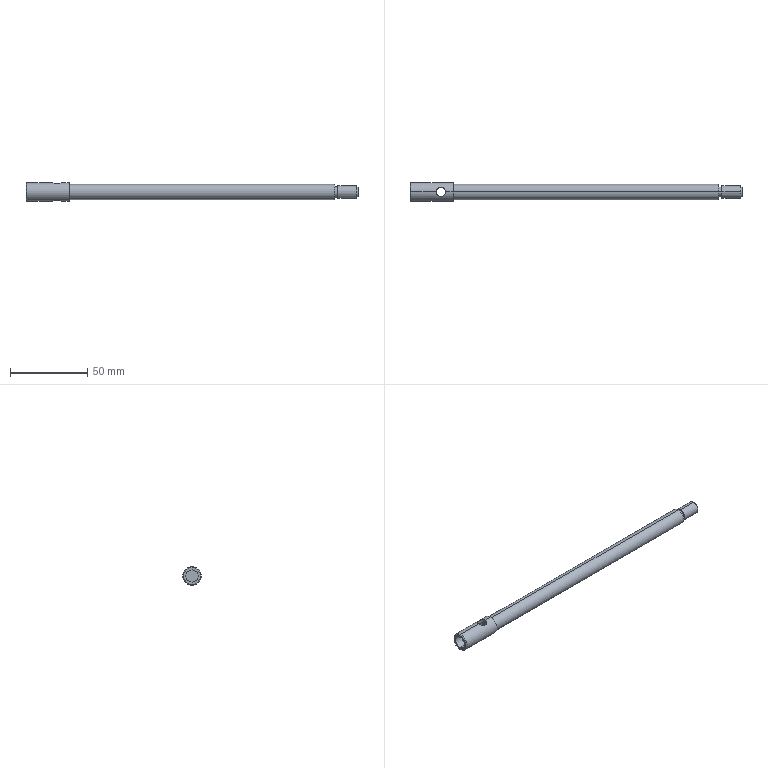Component | SolidWorks | Barrel-1 | 1 solid | 27 faces | box 215 x 12 x 12 mm | volume 14334 mm3 | cylinder 16 | plane 7 | cone 4 | commonest cylinder face diameters 6 x4 8 x4 5 x2 6.5 x2 10 x2 12 x2
STEP:
#1=CARTESIAN_POINT('',(-16.568,1.358,39.941));
#2=VERTEX_POINT('',#1);
#3=CARTESIAN_POINT('',(-16.568,1.358,39.508));
#4=VERTEX_POINT('',#3);
#5=CARTESIAN_POINT('',(-16.568,1.358,39.724));
#6=DIRECTION('',(-1.,0.,0.));
#7=DIRECTION('',(0.,0.,-1.));
#8=AXIS2_PLACEMENT_3D('',#5,#6,#7);
#9=CIRCLE('',#8,0.2165);
#10=EDGE_CURVE('',#2,#4,#9,.T.);
#11=ORIENTED_EDGE('',*,*,#10,.F.);
#12=CARTESIAN_POINT('',(-16.548,1.358,39.961));
#13=VERTEX_POINT('',#12);
#14=CARTESIAN_POINT('',(-16.568,1.358,39.941));
#15=DIRECTION('',(0.7071,0.,0.7071));
#16=VECTOR('',#15,39.37);
#17=LINE('',#14,#16);
#18=EDGE_CURVE('',#2,#13,#17,.T.);
#19=ORIENTED_EDGE('',*,*,#18,.T.);
#20=CARTESIAN_POINT('',(-16.548,1.358,39.488));
#21=VERTEX_POINT('',#20);
#22=CARTESIAN_POINT('',(-16.548,1.358,39.724));
#23=DIRECTION('',(1.,0.,0.));
#24=DIRECTION('',(0.,0.,-1.));
#25=AXIS2_PLACEMENT_3D('',#22,#23,#24);
#26=CIRCLE('',#25,0.2362);
#27=EDGE_CURVE('',#21,#13,#26,.T.);
#28=ORIENTED_EDGE('',*,*,#27,.F.);
#29=CARTESIAN_POINT('',(-16.568,1.358,39.508));
#30=DIRECTION('',(0.7071,0.,-0.7071));
#31=VECTOR('',#30,39.37);
#32=LINE('',#29,#31);
#33=EDGE_CURVE('',#4,#21,#32,.T.);
#34=ORIENTED_EDGE('',*,*,#33,.F.);
#35=EDGE_LOOP('',(#11,#19,#28,#34));
#36=FACE_OUTER_BOUND('',#35,.T.);
#37=CARTESIAN_POINT('',(-16.568,1.358,39.724));
#38=DIRECTION('',(1.,0.,0.));
#39=DIRECTION('',(0.,0.,-1.));
#40=AXIS2_PLACEMENT_3D('',#37,#38,#39);
#41=CONICAL_SURFACE('',#40,0.2165,0.7854);
#42=ADVANCED_FACE('',(#36),#41,.T.);
#43=CARTESIAN_POINT('',(-15.898,1.358,39.961));
#44=VERTEX_POINT('',#43);
#45=CARTESIAN_POINT('',(-15.662,1.358,39.961));
#46=VERTEX_POINT('',#45);
#47=CARTESIAN_POINT('',(-15.898,1.358,39.961));
#48=CARTESIAN_POINT('',(-15.898,1.35,39.961));
#49=CARTESIAN_POINT('',(-15.898,1.342,39.96));
#50=CARTESIAN_POINT('',(-15.894,1.326,39.959));
#51=CARTESIAN_POINT('',(-15.892,1.319,39.958));
#52=CARTESIAN_POINT('',(-15.886,1.305,39.955));
#53=CARTESIAN_POINT('',(-15.882,1.298,39.953));
#54=CARTESIAN_POINT('',(-15.874,1.285,39.949));
#55=CARTESIAN_POINT('',(-15.869,1.279,39.947));
#56=CARTESIAN_POINT('',(-15.858,1.269,39.943));
#57=CARTESIAN_POINT('',(-15.852,1.264,39.941));
#58=CARTESIAN_POINT('',(-15.84,1.255,39.937));
#59=CARTESIAN_POINT('',(-15.833,1.252,39.936));
#60=CARTESIAN_POINT('',(-15.819,1.246,39.932));
#61=CARTESIAN_POINT('',(-15.811,1.243,39.931));
#62=CARTESIAN_POINT('',(-15.796,1.24,39.929));
#63=CARTESIAN_POINT('',(-15.788,1.239,39.929));
#64=CARTESIAN_POINT('',(-15.773,1.239,39.929));
#65=CARTESIAN_POINT('',(-15.765,1.24,39.929));
#66=CARTESIAN_POINT('',(-15.749,1.243,39.931));
#67=CARTESIAN_POINT('',(-15.742,1.246,39.932));
#68=CARTESIAN_POINT('',(-15.72,1.255,39.937));
#69=CARTESIAN_POINT('',(-15.708,1.263,39.941));
#70=CARTESIAN_POINT('',(-15.691,1.279,39.947));
#71=CARTESIAN_POINT('',(-15.687,1.285,39.949));
#72=CARTESIAN_POINT('',(-15.678,1.298,39.953));
#73=CARTESIAN_POINT('',(-15.674,1.305,39.955));
#74=CARTESIAN_POINT('',(-15.668,1.319,39.958));
#75=CARTESIAN_POINT('',(-15.666,1.326,39.959));
#76=CARTESIAN_POINT('',(-15.663,1.342,39.96));
#77=CARTESIAN_POINT('',(-15.662,1.35,39.961));
#78=CARTESIAN_POINT('',(-15.662,1.358,39.961));
#79=B_SPLINE_CURVE_WITH_KNOTS('',3,(#47,#48,#49,#50,#51,#52,#53,#54,#55,#56,#57,#58,#59,#60,#61,#62,#63,#64,#65,#66,#67,#68,#69,#70,#71,#72,#73,#74,#75,#76,#77,#78),.UNSPECIFIED.,.F.,.F.,(4,2,2,2,2,2,2,2,2,2,2,2,2,2,2,4),(0.009543,0.01014,0.01073,0.01133,0.01192,0.01252,0.01312,0.01371,0.01431,0.0149,0.0155,0.01669,0.01728,0.01788,0.01847,0.01907),.UNSPECIFIED.);
#80=EDGE_CURVE('',#44,#46,#79,.T.);
#81=ORIENTED_EDGE('',*,*,#80,.T.);
#82=CARTESIAN_POINT('',(-15.662,1.358,39.882));
#83=VERTEX_POINT('',#82);
#84=CARTESIAN_POINT('',(-15.662,1.358,40.472));
#85=DIRECTION('',(0.,0.,-1.));
#86=VECTOR('',#85,39.37);
#87=LINE('',#84,#86);
#88=EDGE_CURVE('',#46,#83,#87,.T.);
#89=ORIENTED_EDGE('',*,*,#88,.T.);
#90=CARTESIAN_POINT('',(-15.898,1.358,39.882));
#91=VERTEX_POINT('',#90);
#92=CARTESIAN_POINT('',(-15.662,1.358,39.882));
#93=CARTESIAN_POINT('',(-15.662,1.349,39.882));
#94=CARTESIAN_POINT('',(-15.663,1.341,39.881));
#95=CARTESIAN_POINT('',(-15.666,1.326,39.879));
#96=CARTESIAN_POINT('',(-15.669,1.318,39.877));
#97=CARTESIAN_POINT('',(-15.675,1.304,39.873));
#98=CARTESIAN_POINT('',(-15.679,1.297,39.87));
#99=CARTESIAN_POINT('',(-15.687,1.285,39.864));
#100=CARTESIAN_POINT('',(-15.692,1.279,39.861));
#101=CARTESIAN_POINT('',(-15.702,1.268,39.854));
#102=CARTESIAN_POINT('',(-15.708,1.264,39.851));
#103=CARTESIAN_POINT('',(-15.72,1.255,39.844));
#104=CARTESIAN_POINT('',(-15.727,1.252,39.841));
#105=CARTESIAN_POINT('',(-15.741,1.246,39.836));
#106=CARTESIAN_POINT('',(-15.748,1.244,39.833));
#107=CARTESIAN_POINT('',(-15.764,1.24,39.83));
#108=CARTESIAN_POINT('',(-15.772,1.239,39.829));
#109=CARTESIAN_POINT('',(-15.788,1.239,39.829));
#110=CARTESIAN_POINT('',(-15.796,1.24,39.83));
#111=CARTESIAN_POINT('',(-15.812,1.244,39.833));
#112=CARTESIAN_POINT('',(-15.819,1.246,39.836));
#113=CARTESIAN_POINT('',(-15.833,1.252,39.841));
#114=CARTESIAN_POINT('',(-15.84,1.255,39.844));
#115=CARTESIAN_POINT('',(-15.852,1.264,39.851));
#116=CARTESIAN_POINT('',(-15.858,1.268,39.854));
#117=CARTESIAN_POINT('',(-15.869,1.279,39.861));
#118=CARTESIAN_POINT('',(-15.873,1.285,39.864));
#119=CARTESIAN_POINT('',(-15.882,1.297,39.87));
#120=CARTESIAN_POINT('',(-15.886,1.304,39.873));
#121=CARTESIAN_POINT('',(-15.892,1.318,39.877));
#122=CARTESIAN_POINT('',(-15.894,1.326,39.879));
#123=CARTESIAN_POINT('',(-15.898,1.342,39.881));
#124=CARTESIAN_POINT('',(-15.898,1.35,39.882));
#125=CARTESIAN_POINT('',(-15.898,1.358,39.882));
#126=B_SPLINE_CURVE_WITH_KNOTS('',3,(#92,#93,#94,#95,#96,#97,#98,#99,#100,#101,#102,#103,#104,#105,#106,#107,#108,#109,#110,#111,#112,#113,#114,#115,#116,#117,#118,#119,#120,#121,#122,#123,#124,#125),.UNSPECIFIED.,.F.,.F.,(4,2,2,2,2,2,2,2,2,2,2,2,2,2,2,2,4),(0.,0.0006141,0.001228,0.001842,0.002456,0.003071,0.003685,0.004299,0.004913,0.005527,0.006141,0.006755,0.007369,0.007983,0.008598,0.009212,0.009826),.UNSPECIFIED.);
#127=EDGE_CURVE('',#83,#91,#126,.T.);
#128=ORIENTED_EDGE('',*,*,#127,.T.);
#129=CARTESIAN_POINT('',(-15.898,1.358,40.472));
#130=DIRECTION('',(0.,0.,-1.));
#131=VECTOR('',#130,39.37);
#132=LINE('',#129,#131);
#133=EDGE_CURVE('',#44,#91,#132,.T.);
#134=ORIENTED_EDGE('',*,*,#133,.F.);
#135=EDGE_LOOP('',(#81,#89,#128,#134));
#136=FACE_OUTER_BOUND('',#135,.T.);
#137=CARTESIAN_POINT('',(-15.78,1.358,40.472));
#138=DIRECTION('',(0.,0.,-1.));
#139=DIRECTION('',(-1.,0.,0.));
#140=AXIS2_PLACEMENT_3D('',#137,#138,#139);
#141=CYLINDRICAL_SURFACE('',#140,0.1181);
#142=ADVANCED_FACE('',(#136),#141,.F.);
#143=CARTESIAN_POINT('',(-15.898,1.358,39.567));
#144=VERTEX_POINT('',#143);
#145=CARTESIAN_POINT('',(-15.662,1.358,39.567));
#146=VERTEX_POINT('',#145);
#147=CARTESIAN_POINT('',(-15.898,1.358,39.567));
#148=CARTESIAN_POINT('',(-15.898,1.349,39.567));
#149=CARTESIAN_POINT('',(-15.897,1.341,39.568));
#150=CARTESIAN_POINT('',(-15.894,1.326,39.57));
#151=CARTESIAN_POINT('',(-15.892,1.318,39.572));
#152=CARTESIAN_POINT('',(-15.886,1.304,39.576));
#153=CARTESIAN_POINT('',(-15.882,1.297,39.579));
#154=CARTESIAN_POINT('',(-15.873,1.285,39.585));
#155=CARTESIAN_POINT('',(-15.869,1.279,39.588));
#156=CARTESIAN_POINT('',(-15.858,1.268,39.594));
#157=CARTESIAN_POINT('',(-15.852,1.264,39.598));
#158=CARTESIAN_POINT('',(-15.84,1.255,39.604));
#159=CARTESIAN_POINT('',(-15.833,1.252,39.608));
#160=CARTESIAN_POINT('',(-15.819,1.246,39.613));
#161=CARTESIAN_POINT('',(-15.812,1.244,39.616));
#162=CARTESIAN_POINT('',(-15.796,1.24,39.619));
#163=CARTESIAN_POINT('',(-15.788,1.239,39.62));
#164=CARTESIAN_POINT('',(-15.772,1.239,39.62));
#165=CARTESIAN_POINT('',(-15.764,1.24,39.619));
#166=CARTESIAN_POINT('',(-15.748,1.244,39.616));
#167=CARTESIAN_POINT('',(-15.741,1.246,39.613));
#168=CARTESIAN_POINT('',(-15.727,1.252,39.608));
#169=CARTESIAN_POINT('',(-15.72,1.255,39.604));
#170=CARTESIAN_POINT('',(-15.708,1.264,39.598));
#171=CARTESIAN_POINT('',(-15.702,1.268,39.594));
#172=CARTESIAN_POINT('',(-15.692,1.279,39.588));
#173=CARTESIAN_POINT('',(-15.687,1.285,39.585));
#174=CARTESIAN_POINT('',(-15.679,1.297,39.579));
#175=CARTESIAN_POINT('',(-15.675,1.304,39.576));
#176=CARTESIAN_POINT('',(-15.669,1.318,39.572));
#177=CARTESIAN_POINT('',(-15.666,1.326,39.57));
#178=CARTESIAN_POINT('',(-15.663,1.342,39.568));
#179=CARTESIAN_POINT('',(-15.662,1.35,39.567));
#180=CARTESIAN_POINT('',(-15.662,1.358,39.567));
#181=B_SPLINE_CURVE_WITH_KNOTS('',3,(#147,#148,#149,#150,#151,#152,#153,#154,#155,#156,#157,#158,#159,#160,#161,#162,#163,#164,#165,#166,#167,#168,#169,#170,#171,#172,#173,#174,#175,#176,#177,#178,#179,#180),.UNSPECIFIED.,.F.,.F.,(4,2,2,2,2,2,2,2,2,2,2,2,2,2,2,2,4),(0.,0.0006141,0.001228,0.001842,0.002456,0.003071,0.003685,0.004299,0.004913,0.005527,0.006141,0.006755,0.007369,0.007983,0.008598,0.009212,0.009826),.UNSPECIFIED.);
#182=EDGE_CURVE('',#144,#146,#181,.T.);
#183=ORIENTED_EDGE('',*,*,#182,.T.);
#184=CARTESIAN_POINT('',(-15.662,1.358,39.488));
#185=VERTEX_POINT('',#184);
#186=CARTESIAN_POINT('',(-15.662,1.358,40.472));
#187=DIRECTION('',(0.,0.,-1.));
#188=VECTOR('',#187,39.37);
#189=LINE('',#186,#188);
#190=EDGE_CURVE('',#146,#185,#189,.T.);
#191=ORIENTED_EDGE('',*,*,#190,.T.);
#192=CARTESIAN_POINT('',(-15.898,1.358,39.488));
#193=VERTEX_POINT('',#192);
#194=CARTESIAN_POINT('',(-15.662,1.358,39.488));
#195=CARTESIAN_POINT('',(-15.662,1.35,39.488));
#196=CARTESIAN_POINT('',(-15.663,1.342,39.489));
#197=CARTESIAN_POINT('',(-15.666,1.326,39.49));
#198=CARTESIAN_POINT('',(-15.668,1.319,39.491));
#199=CARTESIAN_POINT('',(-15.674,1.305,39.494));
#200=CARTESIAN_POINT('',(-15.678,1.298,39.496));
#201=CARTESIAN_POINT('',(-15.687,1.285,39.499));
#202=CARTESIAN_POINT('',(-15.691,1.279,39.501));
#203=CARTESIAN_POINT('',(-15.702,1.269,39.506));
#204=CARTESIAN_POINT('',(-15.708,1.264,39.508));
#205=CARTESIAN_POINT('',(-15.721,1.255,39.511));
#206=CARTESIAN_POINT('',(-15.728,1.252,39.513));
#207=CARTESIAN_POINT('',(-15.742,1.246,39.516));
#208=CARTESIAN_POINT('',(-15.749,1.243,39.518));
#209=CARTESIAN_POINT('',(-15.764,1.24,39.519));
#210=CARTESIAN_POINT('',(-15.772,1.239,39.52));
#211=CARTESIAN_POINT('',(-15.788,1.239,39.52));
#212=CARTESIAN_POINT('',(-15.796,1.24,39.519));
#213=CARTESIAN_POINT('',(-15.811,1.243,39.518));
#214=CARTESIAN_POINT('',(-15.819,1.246,39.516));
#215=CARTESIAN_POINT('',(-15.84,1.255,39.512));
#216=CARTESIAN_POINT('',(-15.853,1.263,39.508));
#217=CARTESIAN_POINT('',(-15.869,1.279,39.501));
#218=CARTESIAN_POINT('',(-15.874,1.285,39.499));
#219=CARTESIAN_POINT('',(-15.882,1.298,39.496));
#220=CARTESIAN_POINT('',(-15.886,1.305,39.494));
#221=CARTESIAN_POINT('',(-15.892,1.319,39.491));
#222=CARTESIAN_POINT('',(-15.894,1.326,39.49));
#223=CARTESIAN_POINT('',(-15.898,1.342,39.489));
#224=CARTESIAN_POINT('',(-15.898,1.35,39.488));
#225=CARTESIAN_POINT('',(-15.898,1.358,39.488));
#226=B_SPLINE_CURVE_WITH_KNOTS('',3,(#194,#195,#196,#197,#198,#199,#200,#201,#202,#203,#204,#205,#206,#207,#208,#209,#210,#211,#212,#213,#214,#215,#216,#217,#218,#219,#220,#221,#222,#223,#224,#225),.UNSPECIFIED.,.F.,.F.,(4,2,2,2,2,2,2,2,2,2,2,2,2,2,2,4),(0.009543,0.01014,0.01073,0.01133,0.01192,0.01252,0.01312,0.01371,0.01431,0.0149,0.0155,0.01669,0.01728,0.01788,0.01847,0.01907),.UNSPECIFIED.);
#227=EDGE_CURVE('',#185,#193,#226,.T.);
#228=ORIENTED_EDGE('',*,*,#227,.T.);
#229=CARTESIAN_POINT('',(-15.898,1.358,40.472));
#230=DIRECTION('',(0.,0.,-1.));
#231=VECTOR('',#230,39.37);
#232=LINE('',#229,#231);
#233=EDGE_CURVE('',#144,#193,#232,.T.);
#234=ORIENTED_EDGE('',*,*,#233,.F.);
#235=EDGE_LOOP('',(#183,#191,#228,#234));
#236=FACE_OUTER_BOUND('',#235,.T.);
#237=CARTESIAN_POINT('',(-15.78,1.358,40.472));
#238=DIRECTION('',(0.,0.,-1.));
#239=DIRECTION('',(-1.,0.,0.));
#240=AXIS2_PLACEMENT_3D('',#237,#238,#239);
#241=CYLINDRICAL_SURFACE('',#240,0.1181);
#242=ADVANCED_FACE('',(#236),#241,.F.);
#243=CARTESIAN_POINT('',(-8.103,1.358,39.606));
#244=VERTEX_POINT('',#243);
#245=CARTESIAN_POINT('',(-8.103,1.358,39.843));
#246=VERTEX_POINT('',#245);
#247=CARTESIAN_POINT('',(-8.103,1.358,39.724));
#248=DIRECTION('',(1.,0.,0.));
#249=DIRECTION('',(0.,0.,1.));
#250=AXIS2_PLACEMENT_3D('',#247,#248,#249);
#251=CIRCLE('',#250,0.1181);
#252=EDGE_CURVE('',#244,#246,#251,.T.);
#253=ORIENTED_EDGE('',*,*,#252,.F.);
#254=CARTESIAN_POINT('',(-8.142,1.358,39.567));
#255=VERTEX_POINT('',#254);
#256=CARTESIAN_POINT('',(-8.142,1.358,39.567));
#257=DIRECTION('',(-0.7071,0.,-0.7071));
#258=VECTOR('',#257,39.37);
#259=LINE('',#256,#258);
#260=EDGE_CURVE('',#244,#255,#259,.T.);
#261=ORIENTED_EDGE('',*,*,#260,.T.);
#262=CARTESIAN_POINT('',(-8.142,1.358,39.882));
#263=VERTEX_POINT('',#262);
#264=CARTESIAN_POINT('',(-8.142,1.358,39.724));
#265=DIRECTION('',(-1.,0.,0.));
#266=DIRECTION('',(0.,0.,1.));
#267=AXIS2_PLACEMENT_3D('',#264,#265,#266);
#268=CIRCLE('',#267,0.1575);
#269=EDGE_CURVE('',#263,#255,#268,.T.);
#270=ORIENTED_EDGE('',*,*,#269,.F.);
#271=CARTESIAN_POINT('',(-8.142,1.358,39.882));
#272=DIRECTION('',(-0.7071,0.,0.7071));
#273=VECTOR('',#272,39.37);
#274=LINE('',#271,#273);
#275=EDGE_CURVE('',#246,#263,#274,.T.);
#276=ORIENTED_EDGE('',*,*,#275,.F.);
#277=EDGE_LOOP('',(#253,#261,#270,#276));
#278=FACE_OUTER_BOUND('',#277,.T.);
#279=CARTESIAN_POINT('',(-8.142,1.358,39.724));
#280=DIRECTION('',(-1.,0.,0.));
#281=DIRECTION('',(0.,0.,1.));
#282=AXIS2_PLACEMENT_3D('',#279,#280,#281);
#283=CONICAL_SURFACE('',#282,0.1575,0.7854);
#284=ADVANCED_FACE('',(#278),#283,.T.);
#285=CARTESIAN_POINT('',(-11.45,1.358,39.823));
#286=VERTEX_POINT('',#285);
#287=CARTESIAN_POINT('',(-11.45,1.358,39.626));
#288=VERTEX_POINT('',#287);
#289=CARTESIAN_POINT('',(-11.45,1.358,39.724));
#290=DIRECTION('',(1.,0.,0.));
#291=DIRECTION('',(0.,0.,-1.));
#292=AXIS2_PLACEMENT_3D('',#289,#290,#291);
#293=CIRCLE('',#292,0.09843);
#294=EDGE_CURVE('',#286,#288,#293,.T.);
#295=ORIENTED_EDGE('',*,*,#294,.F.);
#296=CARTESIAN_POINT('',(-8.103,1.358,39.823));
#297=VERTEX_POINT('',#296);
#298=CARTESIAN_POINT('',(-11.45,1.358,39.823));
#299=DIRECTION('',(1.,0.,0.));
#300=VECTOR('',#299,39.37);
#301=LINE('',#298,#300);
#302=EDGE_CURVE('',#286,#297,#301,.T.);
#303=ORIENTED_EDGE('',*,*,#302,.T.);
#304=CARTESIAN_POINT('',(-8.103,1.358,39.626));
#305=VERTEX_POINT('',#304);
#306=CARTESIAN_POINT('',(-8.103,1.358,39.724));
#307=DIRECTION('',(1.,0.,0.));
#308=DIRECTION('',(0.,0.,-1.));
#309=AXIS2_PLACEMENT_3D('',#306,#307,#308);
#310=CIRCLE('',#309,0.09843);
#311=EDGE_CURVE('',#297,#305,#310,.T.);
#312=ORIENTED_EDGE('',*,*,#311,.T.);
#313=CARTESIAN_POINT('',(-11.45,1.358,39.626));
#314=DIRECTION('',(1.,0.,0.));
#315=VECTOR('',#314,39.37);
#316=LINE('',#313,#315);
#317=EDGE_CURVE('',#288,#305,#316,.T.);
#318=ORIENTED_EDGE('',*,*,#317,.F.);
#319=EDGE_LOOP('',(#295,#303,#312,#318));
#320=FACE_OUTER_BOUND('',#319,.T.);
#321=CARTESIAN_POINT('',(-11.45,1.358,39.724));
#322=DIRECTION('',(1.,0.,0.));
#323=DIRECTION('',(0.,0.,-1.));
#324=AXIS2_PLACEMENT_3D('',#321,#322,#323);
#325=CYLINDRICAL_SURFACE('',#324,0.09843);
#326=ADVANCED_FACE('',(#320),#325,.F.);
#327=ORIENTED_EDGE('',*,*,#269,.T.);
#328=CARTESIAN_POINT('',(-8.615,1.358,39.567));
#329=VERTEX_POINT('',#328);
#330=CARTESIAN_POINT('',(-16.568,1.358,39.567));
#331=DIRECTION('',(-1.,0.,0.));
#332=VECTOR('',#331,39.37);
#333=LINE('',#330,#332);
#334=EDGE_CURVE('',#255,#329,#333,.T.);
#335=ORIENTED_EDGE('',*,*,#334,.T.);
#336=CARTESIAN_POINT('',(-8.615,1.358,39.882));
#337=VERTEX_POINT('',#336);
#338=CARTESIAN_POINT('',(-8.615,1.358,39.724));
#339=DIRECTION('',(-1.,0.,0.));
#340=DIRECTION('',(0.,0.,1.));
#341=AXIS2_PLACEMENT_3D('',#338,#339,#340);
#342=CIRCLE('',#341,0.1575);
#343=EDGE_CURVE('',#337,#329,#342,.T.);
#344=ORIENTED_EDGE('',*,*,#343,.F.);
#345=CARTESIAN_POINT('',(-16.568,1.358,39.882));
#346=DIRECTION('',(-1.,0.,0.));
#347=VECTOR('',#346,39.37);
#348=LINE('',#345,#347);
#349=EDGE_CURVE('',#263,#337,#348,.T.);
#350=ORIENTED_EDGE('',*,*,#349,.F.);
#351=EDGE_LOOP('',(#327,#335,#344,#350));
#352=FACE_OUTER_BOUND('',#351,.T.);
#353=CARTESIAN_POINT('',(-16.568,1.358,39.724));
#354=DIRECTION('',(-1.,0.,0.));
#355=DIRECTION('',(0.,0.,1.));
#356=AXIS2_PLACEMENT_3D('',#353,#354,#355);
#357=CYLINDRICAL_SURFACE('',#356,0.1575);
#358=ADVANCED_FACE('',(#352),#357,.T.);
#359=CARTESIAN_POINT('',(-8.615,1.358,39.852));
#360=VERTEX_POINT('',#359);
#361=CARTESIAN_POINT('',(-8.615,1.358,39.596));
#362=VERTEX_POINT('',#361);
#363=CARTESIAN_POINT('',(-8.615,1.358,39.724));
#364=DIRECTION('',(-1.,0.,0.));
#365=DIRECTION('',(0.,0.,1.));
#366=AXIS2_PLACEMENT_3D('',#363,#364,#365);
#367=CIRCLE('',#366,0.128);
#368=EDGE_CURVE('',#360,#362,#367,.T.);
#369=ORIENTED_EDGE('',*,*,#368,.T.);
#370=CARTESIAN_POINT('',(-8.694,1.358,39.596));
#371=VERTEX_POINT('',#370);
#372=CARTESIAN_POINT('',(-16.568,1.358,39.596));
#373=DIRECTION('',(-1.,0.,0.));
#374=VECTOR('',#373,39.37);
#375=LINE('',#372,#374);
#376=EDGE_CURVE('',#362,#371,#375,.T.);
#377=ORIENTED_EDGE('',*,*,#376,.T.);
#378=CARTESIAN_POINT('',(-8.694,1.358,39.852));
#379=VERTEX_POINT('',#378);
#380=CARTESIAN_POINT('',(-8.694,1.358,39.724));
#381=DIRECTION('',(-1.,0.,0.));
#382=DIRECTION('',(0.,0.,1.));
#383=AXIS2_PLACEMENT_3D('',#380,#381,#382);
#384=CIRCLE('',#383,0.128);
#385=EDGE_CURVE('',#379,#371,#384,.T.);
#386=ORIENTED_EDGE('',*,*,#385,.F.);
#387=CARTESIAN_POINT('',(-16.568,1.358,39.852));
#388=DIRECTION('',(-1.,0.,0.));
#389=VECTOR('',#388,39.37);
#390=LINE('',#387,#389);
#391=EDGE_CURVE('',#360,#379,#390,.T.);
#392=ORIENTED_EDGE('',*,*,#391,.F.);
#393=EDGE_LOOP('',(#369,#377,#386,#392));
#394=FACE_OUTER_BOUND('',#393,.T.);
#395=CARTESIAN_POINT('',(-16.568,1.358,39.724));
#396=DIRECTION('',(-1.,0.,0.));
#397=DIRECTION('',(0.,0.,1.));
#398=AXIS2_PLACEMENT_3D('',#395,#396,#397);
#399=CYLINDRICAL_SURFACE('',#398,0.128);
#400=ADVANCED_FACE('',(#394),#399,.T.);
#401=CARTESIAN_POINT('',(-8.694,1.358,39.921));
#402=VERTEX_POINT('',#401);
#403=CARTESIAN_POINT('',(-8.694,1.358,39.528));
#404=VERTEX_POINT('',#403);
#405=CARTESIAN_POINT('',(-8.694,1.358,39.724));
#406=DIRECTION('',(-1.,0.,0.));
#407=DIRECTION('',(0.,0.,1.));
#408=AXIS2_PLACEMENT_3D('',#405,#406,#407);
#409=CIRCLE('',#408,0.1969);
#410=EDGE_CURVE('',#402,#404,#409,.T.);
#411=ORIENTED_EDGE('',*,*,#410,.T.);
#412=CARTESIAN_POINT('',(-15.465,1.358,39.528));
#413=VERTEX_POINT('',#412);
#414=CARTESIAN_POINT('',(-16.568,1.358,39.528));
#415=DIRECTION('',(-1.,0.,0.));
#416=VECTOR('',#415,39.37);
#417=LINE('',#414,#416);
#418=EDGE_CURVE('',#404,#413,#417,.T.);
#419=ORIENTED_EDGE('',*,*,#418,.T.);
#420=CARTESIAN_POINT('',(-15.465,1.358,39.921));
#421=VERTEX_POINT('',#420);
#422=CARTESIAN_POINT('',(-15.465,1.358,39.724));
#423=DIRECTION('',(-1.,0.,0.));
#424=DIRECTION('',(0.,0.,1.));
#425=AXIS2_PLACEMENT_3D('',#422,#423,#424);
#426=CIRCLE('',#425,0.1969);
#427=EDGE_CURVE('',#421,#413,#426,.T.);
#428=ORIENTED_EDGE('',*,*,#427,.F.);
#429=CARTESIAN_POINT('',(-16.568,1.358,39.921));
#430=DIRECTION('',(-1.,0.,0.));
#431=VECTOR('',#430,39.37);
#432=LINE('',#429,#431);
#433=EDGE_CURVE('',#402,#421,#432,.T.);
#434=ORIENTED_EDGE('',*,*,#433,.F.);
#435=EDGE_LOOP('',(#411,#419,#428,#434));
#436=FACE_OUTER_BOUND('',#435,.T.);
#437=CARTESIAN_POINT('',(-16.568,1.358,39.724));
#438=DIRECTION('',(-1.,0.,0.));
#439=DIRECTION('',(0.,0.,1.));
#440=AXIS2_PLACEMENT_3D('',#437,#438,#439);
#441=CYLINDRICAL_SURFACE('',#440,0.1969);
#442=ADVANCED_FACE('',(#436),#441,.T.);
#443=CARTESIAN_POINT('',(-15.583,1.358,39.567));
#444=VERTEX_POINT('',#443);
#445=CARTESIAN_POINT('',(-15.583,1.358,39.882));
#446=VERTEX_POINT('',#445);
#447=CARTESIAN_POINT('',(-15.583,1.358,39.724));
#448=DIRECTION('',(-1.,0.,0.));
#449=DIRECTION('',(0.,0.,1.));
#450=AXIS2_PLACEMENT_3D('',#447,#448,#449);
#451=CIRCLE('',#450,0.1575);
#452=EDGE_CURVE('',#444,#446,#451,.T.);
#453=ORIENTED_EDGE('',*,*,#452,.F.);
#454=CARTESIAN_POINT('',(-15.583,1.358,39.567));
#455=DIRECTION('',(-1.,0.,0.));
#456=VECTOR('',#455,39.37);
#457=LINE('',#454,#456);
#458=EDGE_CURVE('',#444,#146,#457,.T.);
#459=ORIENTED_EDGE('',*,*,#458,.T.);
#460=ORIENTED_EDGE('',*,*,#182,.F.);
#461=CARTESIAN_POINT('',(-16.568,1.358,39.567));
#462=VERTEX_POINT('',#461);
#463=CARTESIAN_POINT('',(-15.583,1.358,39.567));
#464=DIRECTION('',(-1.,0.,0.));
#465=VECTOR('',#464,39.37);
#466=LINE('',#463,#465);
#467=EDGE_CURVE('',#144,#462,#466,.T.);
#468=ORIENTED_EDGE('',*,*,#467,.T.);
#469=CARTESIAN_POINT('',(-16.568,1.358,39.882));
#470=VERTEX_POINT('',#469);
#471=CARTESIAN_POINT('',(-16.568,1.358,39.724));
#472=DIRECTION('',(-1.,0.,0.));
#473=DIRECTION('',(0.,0.,1.));
#474=AXIS2_PLACEMENT_3D('',#471,#472,#473);
#475=CIRCLE('',#474,0.1575);
#476=EDGE_CURVE('',#462,#470,#475,.T.);
#477=ORIENTED_EDGE('',*,*,#476,.T.);
#478=CARTESIAN_POINT('',(-15.583,1.358,39.882));
#479=DIRECTION('',(-1.,0.,0.));
#480=VECTOR('',#479,39.37);
#481=LINE('',#478,#480);
#482=EDGE_CURVE('',#91,#470,#481,.T.);
#483=ORIENTED_EDGE('',*,*,#482,.F.);
#484=ORIENTED_EDGE('',*,*,#127,.F.);
#485=CARTESIAN_POINT('',(-15.583,1.358,39.882));
#486=DIRECTION('',(-1.,0.,0.));
#487=VECTOR('',#486,39.37);
#488=LINE('',#485,#487);
#489=EDGE_CURVE('',#446,#83,#488,.T.);
#490=ORIENTED_EDGE('',*,*,#489,.F.);
#491=EDGE_LOOP('',(#453,#459,#460,#468,#477,#483,#484,#490));
#492=FACE_OUTER_BOUND('',#491,.T.);
#493=CARTESIAN_POINT('',(-15.583,1.358,39.724));
#494=DIRECTION('',(-1.,0.,0.));
#495=DIRECTION('',(0.,0.,1.));
#496=AXIS2_PLACEMENT_3D('',#493,#494,#495);
#497=CYLINDRICAL_SURFACE('',#496,0.1575);
#498=ADVANCED_FACE('',(#492),#497,.F.);
#499=CARTESIAN_POINT('',(-15.465,1.358,39.961));
#500=VERTEX_POINT('',#499);
#501=CARTESIAN_POINT('',(-15.465,1.358,39.488));
#502=VERTEX_POINT('',#501);
#503=CARTESIAN_POINT('',(-15.465,1.358,39.724));
#504=DIRECTION('',(-1.,0.,0.));
#505=DIRECTION('',(0.,0.,1.));
#506=AXIS2_PLACEMENT_3D('',#503,#504,#505);
#507=CIRCLE('',#506,0.2362);
#508=EDGE_CURVE('',#500,#502,#507,.T.);
#509=ORIENTED_EDGE('',*,*,#508,.T.);
#510=CARTESIAN_POINT('',(-16.568,1.358,39.488));
#511=DIRECTION('',(-1.,0.,0.));
#512=VECTOR('',#511,39.37);
#513=LINE('',#510,#512);
#514=EDGE_CURVE('',#502,#185,#513,.T.);
#515=ORIENTED_EDGE('',*,*,#514,.T.);
#516=CARTESIAN_POINT('',(-15.898,1.358,39.488));
#517=CARTESIAN_POINT('',(-15.898,1.366,39.488));
#518=CARTESIAN_POINT('',(-15.898,1.373,39.489));
#519=CARTESIAN_POINT('',(-15.894,1.389,39.49));
#520=CARTESIAN_POINT('',(-15.892,1.396,39.491));
#521=CARTESIAN_POINT('',(-15.886,1.41,39.494));
#522=CARTESIAN_POINT('',(-15.882,1.417,39.496));
#523=CARTESIAN_POINT('',(-15.874,1.43,39.499));
#524=CARTESIAN_POINT('',(-15.869,1.436,39.501));
#525=CARTESIAN_POINT('',(-15.858,1.447,39.506));
#526=CARTESIAN_POINT('',(-15.852,1.451,39.508));
#527=CARTESIAN_POINT('',(-15.84,1.46,39.511));
#528=CARTESIAN_POINT('',(-15.833,1.464,39.513));
#529=CARTESIAN_POINT('',(-15.819,1.469,39.516));
#530=CARTESIAN_POINT('',(-15.811,1.472,39.518));
#531=CARTESIAN_POINT('',(-15.796,1.475,39.519));
#532=CARTESIAN_POINT('',(-15.788,1.476,39.52));
#533=CARTESIAN_POINT('',(-15.772,1.476,39.52));
#534=CARTESIAN_POINT('',(-15.765,1.475,39.519));
#535=CARTESIAN_POINT('',(-15.749,1.472,39.518));
#536=CARTESIAN_POINT('',(-15.742,1.47,39.516));
#537=CARTESIAN_POINT('',(-15.727,1.464,39.513));
#538=CARTESIAN_POINT('',(-15.721,1.46,39.511));
#539=CARTESIAN_POINT('',(-15.708,1.451,39.508));
#540=CARTESIAN_POINT('',(-15.702,1.446,39.505));
#541=CARTESIAN_POINT('',(-15.691,1.436,39.501));
#542=CARTESIAN_POINT('',(-15.687,1.43,39.499));
#543=CARTESIAN_POINT('',(-15.678,1.417,39.496));
#544=CARTESIAN_POINT('',(-15.674,1.41,39.494));
#545=CARTESIAN_POINT('',(-15.668,1.396,39.491));
#546=CARTESIAN_POINT('',(-15.666,1.389,39.49));
#547=CARTESIAN_POINT('',(-15.663,1.373,39.489));
#548=CARTESIAN_POINT('',(-15.662,1.365,39.488));
#549=CARTESIAN_POINT('',(-15.662,1.358,39.488));
#550=B_SPLINE_CURVE_WITH_KNOTS('',3,(#516,#517,#518,#519,#520,#521,#522,#523,#524,#525,#526,#527,#528,#529,#530,#531,#532,#533,#534,#535,#536,#537,#538,#539,#540,#541,#542,#543,#544,#545,#546,#547,#548,#549),.UNSPECIFIED.,.F.,.F.,(4,2,2,2,2,2,2,2,2,2,2,2,2,2,2,2,4),(0.,0.0005964,0.001193,0.001789,0.002386,0.002982,0.003579,0.004175,0.004771,0.005368,0.005964,0.006561,0.007157,0.007754,0.00835,0.008947,0.009543),.UNSPECIFIED.);
#551=EDGE_CURVE('',#193,#185,#550,.T.);
#552=ORIENTED_EDGE('',*,*,#551,.F.);
#553=CARTESIAN_POINT('',(-16.568,1.358,39.488));
#554=DIRECTION('',(-1.,0.,0.));
#555=VECTOR('',#554,39.37);
#556=LINE('',#553,#555);
#557=EDGE_CURVE('',#193,#21,#556,.T.);
#558=ORIENTED_EDGE('',*,*,#557,.T.);
#559=ORIENTED_EDGE('',*,*,#27,.T.);
#560=CARTESIAN_POINT('',(-16.568,1.358,39.961));
#561=DIRECTION('',(-1.,0.,0.));
#562=VECTOR('',#561,39.37);
#563=LINE('',#560,#562);
#564=EDGE_CURVE('',#44,#13,#563,.T.);
#565=ORIENTED_EDGE('',*,*,#564,.F.);
#566=CARTESIAN_POINT('',(-15.662,1.358,39.961));
#567=CARTESIAN_POINT('',(-15.662,1.366,39.961));
#568=CARTESIAN_POINT('',(-15.663,1.373,39.96));
#569=CARTESIAN_POINT('',(-15.666,1.389,39.959));
#570=CARTESIAN_POINT('',(-15.668,1.396,39.958));
#571=CARTESIAN_POINT('',(-15.674,1.41,39.955));
#572=CARTESIAN_POINT('',(-15.678,1.417,39.953));
#573=CARTESIAN_POINT('',(-15.687,1.43,39.949));
#574=CARTESIAN_POINT('',(-15.691,1.436,39.947));
#575=CARTESIAN_POINT('',(-15.702,1.447,39.943));
#576=CARTESIAN_POINT('',(-15.708,1.451,39.941));
#577=CARTESIAN_POINT('',(-15.721,1.46,39.937));
#578=CARTESIAN_POINT('',(-15.727,1.464,39.936));
#579=CARTESIAN_POINT('',(-15.742,1.469,39.932));
#580=CARTESIAN_POINT('',(-15.749,1.472,39.931));
#581=CARTESIAN_POINT('',(-15.764,1.475,39.929));
#582=CARTESIAN_POINT('',(-15.772,1.476,39.929));
#583=CARTESIAN_POINT('',(-15.788,1.476,39.929));
#584=CARTESIAN_POINT('',(-15.796,1.475,39.929));
#585=CARTESIAN_POINT('',(-15.811,1.472,39.931));
#586=CARTESIAN_POINT('',(-15.819,1.47,39.932));
#587=CARTESIAN_POINT('',(-15.833,1.464,39.936));
#588=CARTESIAN_POINT('',(-15.84,1.46,39.937));
#589=CARTESIAN_POINT('',(-15.852,1.451,39.941));
#590=CARTESIAN_POINT('',(-15.858,1.446,39.943));
#591=CARTESIAN_POINT('',(-15.869,1.436,39.947));
#592=CARTESIAN_POINT('',(-15.874,1.43,39.949));
#593=CARTESIAN_POINT('',(-15.883,1.417,39.953));
#594=CARTESIAN_POINT('',(-15.886,1.41,39.955));
#595=CARTESIAN_POINT('',(-15.892,1.396,39.958));
#596=CARTESIAN_POINT('',(-15.894,1.389,39.959));
#597=CARTESIAN_POINT('',(-15.898,1.373,39.96));
#598=CARTESIAN_POINT('',(-15.898,1.365,39.961));
#599=CARTESIAN_POINT('',(-15.898,1.358,39.961));
#600=B_SPLINE_CURVE_WITH_KNOTS('',3,(#566,#567,#568,#569,#570,#571,#572,#573,#574,#575,#576,#577,#578,#579,#580,#581,#582,#583,#584,#585,#586,#587,#588,#589,#590,#591,#592,#593,#594,#595,#596,#597,#598,#599),.UNSPECIFIED.,.F.,.F.,(4,2,2,2,2,2,2,2,2,2,2,2,2,2,2,2,4),(0.,0.0005964,0.001193,0.001789,0.002386,0.002982,0.003579,0.004175,0.004771,0.005368,0.005964,0.006561,0.007157,0.007754,0.00835,0.008947,0.009543),.UNSPECIFIED.);
#601=EDGE_CURVE('',#46,#44,#600,.T.);
#602=ORIENTED_EDGE('',*,*,#601,.F.);
#603=CARTESIAN_POINT('',(-16.568,1.358,39.961));
#604=DIRECTION('',(-1.,0.,0.));
#605=VECTOR('',#604,39.37);
#606=LINE('',#603,#605);
#607=EDGE_CURVE('',#500,#46,#606,.T.);
#608=ORIENTED_EDGE('',*,*,#607,.F.);
#609=EDGE_LOOP('',(#509,#515,#552,#558,#559,#565,#602,#608));
#610=FACE_OUTER_BOUND('',#609,.T.);
#611=CARTESIAN_POINT('',(-16.568,1.358,39.724));
#612=DIRECTION('',(-1.,0.,0.));
#613=DIRECTION('',(0.,0.,1.));
#614=AXIS2_PLACEMENT_3D('',#611,#612,#613);
#615=CYLINDRICAL_SURFACE('',#614,0.2362);
#616=ADVANCED_FACE('',(#610),#615,.T.);
#617=ORIENTED_EDGE('',*,*,#514,.F.);
#618=CARTESIAN_POINT('',(-15.465,1.358,39.724));
#619=DIRECTION('',(-1.,0.,0.));
#620=DIRECTION('',(0.,0.,1.));
#621=AXIS2_PLACEMENT_3D('',#618,#619,#620);
#622=CIRCLE('',#621,0.2362);
#623=EDGE_CURVE('',#502,#500,#622,.T.);
#624=ORIENTED_EDGE('',*,*,#623,.T.);
#625=ORIENTED_EDGE('',*,*,#607,.T.);
#626=ORIENTED_EDGE('',*,*,#80,.F.);
#627=ORIENTED_EDGE('',*,*,#564,.T.);
#628=CARTESIAN_POINT('',(-16.548,1.358,39.724));
#629=DIRECTION('',(1.,0.,0.));
#630=DIRECTION('',(0.,0.,-1.));
#631=AXIS2_PLACEMENT_3D('',#628,#629,#630);
#632=CIRCLE('',#631,0.2362);
#633=EDGE_CURVE('',#13,#21,#632,.T.);
#634=ORIENTED_EDGE('',*,*,#633,.T.);
#635=ORIENTED_EDGE('',*,*,#557,.F.);
#636=ORIENTED_EDGE('',*,*,#227,.F.);
#637=EDGE_LOOP('',(#617,#624,#625,#626,#627,#634,#635,#636));
#638=FACE_OUTER_BOUND('',#637,.T.);
#639=CARTESIAN_POINT('',(-16.568,1.358,39.724));
#640=DIRECTION('',(-1.,0.,0.));
#641=DIRECTION('',(0.,0.,1.));
#642=AXIS2_PLACEMENT_3D('',#639,#640,#641);
#643=CYLINDRICAL_SURFACE('',#642,0.2362);
#644=ADVANCED_FACE('',(#638),#643,.T.);
#645=ORIENTED_EDGE('',*,*,#458,.F.);
#646=CARTESIAN_POINT('',(-15.583,1.358,39.724));
#647=DIRECTION('',(-1.,0.,0.));
#648=DIRECTION('',(0.,0.,1.));
#649=AXIS2_PLACEMENT_3D('',#646,#647,#648);
#650=CIRCLE('',#649,0.1575);
#651=EDGE_CURVE('',#446,#444,#650,.T.);
#652=ORIENTED_EDGE('',*,*,#651,.F.);
#653=ORIENTED_EDGE('',*,*,#489,.T.);
#654=CARTESIAN_POINT('',(-15.898,1.358,39.882));
#655=CARTESIAN_POINT('',(-15.898,1.366,39.882));
#656=CARTESIAN_POINT('',(-15.897,1.374,39.881));
#657=CARTESIAN_POINT('',(-15.894,1.39,39.879));
#658=CARTESIAN_POINT('',(-15.892,1.397,39.877));
#659=CARTESIAN_POINT('',(-15.883,1.419,39.87));
#660=CARTESIAN_POINT('',(-15.874,1.431,39.864));
#661=CARTESIAN_POINT('',(-15.858,1.447,39.854));
#662=CARTESIAN_POINT('',(-15.852,1.452,39.851));
#663=CARTESIAN_POINT('',(-15.84,1.46,39.844));
#664=CARTESIAN_POINT('',(-15.833,1.463,39.841));
#665=CARTESIAN_POINT('',(-15.82,1.469,39.836));
#666=CARTESIAN_POINT('',(-15.812,1.472,39.833));
#667=CARTESIAN_POINT('',(-15.8,1.474,39.83));
#668=CARTESIAN_POINT('',(-15.796,1.475,39.83));
#669=CARTESIAN_POINT('',(-15.788,1.475,39.829));
#670=CARTESIAN_POINT('',(-15.784,1.476,39.829));
#671=CARTESIAN_POINT('',(-15.772,1.476,39.829));
#672=CARTESIAN_POINT('',(-15.764,1.475,39.83));
#673=CARTESIAN_POINT('',(-15.748,1.472,39.833));
#674=CARTESIAN_POINT('',(-15.741,1.469,39.836));
#675=CARTESIAN_POINT('',(-15.727,1.463,39.841));
#676=CARTESIAN_POINT('',(-15.72,1.46,39.844));
#677=CARTESIAN_POINT('',(-15.708,1.451,39.851));
#678=CARTESIAN_POINT('',(-15.703,1.447,39.854));
#679=CARTESIAN_POINT('',(-15.692,1.436,39.861));
#680=CARTESIAN_POINT('',(-15.687,1.431,39.864));
#681=CARTESIAN_POINT('',(-15.679,1.418,39.87));
#682=CARTESIAN_POINT('',(-15.675,1.412,39.873));
#683=CARTESIAN_POINT('',(-15.669,1.397,39.877));
#684=CARTESIAN_POINT('',(-15.666,1.39,39.879));
#685=CARTESIAN_POINT('',(-15.663,1.374,39.881));
#686=CARTESIAN_POINT('',(-15.662,1.366,39.882));
#687=CARTESIAN_POINT('',(-15.662,1.358,39.882));
#688=B_SPLINE_CURVE_WITH_KNOTS('',3,(#654,#655,#656,#657,#658,#659,#660,#661,#662,#663,#664,#665,#666,#667,#668,#669,#670,#671,#672,#673,#674,#675,#676,#677,#678,#679,#680,#681,#682,#683,#684,#685,#686,#687),.UNSPECIFIED.,.F.,.F.,(4,2,2,2,2,2,2,2,2,2,2,2,2,2,2,2,4),(0.009826,0.01044,0.01105,0.01228,0.01289,0.0135,0.01412,0.01442,0.01473,0.01534,0.01595,0.01657,0.01718,0.01779,0.01841,0.01902,0.01963),.UNSPECIFIED.);
#689=EDGE_CURVE('',#91,#83,#688,.T.);
#690=ORIENTED_EDGE('',*,*,#689,.F.);
#691=ORIENTED_EDGE('',*,*,#482,.T.);
#692=CARTESIAN_POINT('',(-16.568,1.358,39.724));
#693=DIRECTION('',(-1.,0.,0.));
#694=DIRECTION('',(0.,0.,1.));
#695=AXIS2_PLACEMENT_3D('',#692,#693,#694);
#696=CIRCLE('',#695,0.1575);
#697=EDGE_CURVE('',#470,#462,#696,.T.);
#698=ORIENTED_EDGE('',*,*,#697,.T.);
#699=ORIENTED_EDGE('',*,*,#467,.F.);
#700=CARTESIAN_POINT('',(-15.662,1.358,39.567));
#701=CARTESIAN_POINT('',(-15.662,1.366,39.567));
#702=CARTESIAN_POINT('',(-15.663,1.374,39.568));
#703=CARTESIAN_POINT('',(-15.666,1.39,39.57));
#704=CARTESIAN_POINT('',(-15.669,1.397,39.572));
#705=CARTESIAN_POINT('',(-15.678,1.419,39.578));
#706=CARTESIAN_POINT('',(-15.687,1.431,39.585));
#707=CARTESIAN_POINT('',(-15.702,1.447,39.594));
#708=CARTESIAN_POINT('',(-15.708,1.452,39.598));
#709=CARTESIAN_POINT('',(-15.721,1.46,39.604));
#710=CARTESIAN_POINT('',(-15.727,1.463,39.608));
#711=CARTESIAN_POINT('',(-15.741,1.469,39.613));
#712=CARTESIAN_POINT('',(-15.748,1.472,39.616));
#713=CARTESIAN_POINT('',(-15.76,1.474,39.618));
#714=CARTESIAN_POINT('',(-15.764,1.475,39.619));
#715=CARTESIAN_POINT('',(-15.772,1.475,39.62));
#716=CARTESIAN_POINT('',(-15.776,1.476,39.62));
#717=CARTESIAN_POINT('',(-15.788,1.476,39.62));
#718=CARTESIAN_POINT('',(-15.796,1.475,39.619));
#719=CARTESIAN_POINT('',(-15.812,1.472,39.616));
#720=CARTESIAN_POINT('',(-15.819,1.469,39.613));
#721=CARTESIAN_POINT('',(-15.833,1.463,39.608));
#722=CARTESIAN_POINT('',(-15.84,1.46,39.604));
#723=CARTESIAN_POINT('',(-15.852,1.451,39.598));
#724=CARTESIAN_POINT('',(-15.858,1.447,39.595));
#725=CARTESIAN_POINT('',(-15.868,1.436,39.588));
#726=CARTESIAN_POINT('',(-15.873,1.431,39.585));
#727=CARTESIAN_POINT('',(-15.882,1.418,39.579));
#728=CARTESIAN_POINT('',(-15.886,1.412,39.576));
#729=CARTESIAN_POINT('',(-15.892,1.397,39.572));
#730=CARTESIAN_POINT('',(-15.894,1.39,39.57));
#731=CARTESIAN_POINT('',(-15.897,1.374,39.568));
#732=CARTESIAN_POINT('',(-15.898,1.366,39.567));
#733=CARTESIAN_POINT('',(-15.898,1.358,39.567));
#734=B_SPLINE_CURVE_WITH_KNOTS('',3,(#700,#701,#702,#703,#704,#705,#706,#707,#708,#709,#710,#711,#712,#713,#714,#715,#716,#717,#718,#719,#720,#721,#722,#723,#724,#725,#726,#727,#728,#729,#730,#731,#732,#733),.UNSPECIFIED.,.F.,.F.,(4,2,2,2,2,2,2,2,2,2,2,2,2,2,2,2,4),(0.009826,0.01044,0.01105,0.01228,0.01289,0.0135,0.01412,0.01442,0.01473,0.01534,0.01595,0.01657,0.01718,0.01779,0.01841,0.01902,0.01963),.UNSPECIFIED.);
#735=EDGE_CURVE('',#146,#144,#734,.T.);
#736=ORIENTED_EDGE('',*,*,#735,.F.);
#737=EDGE_LOOP('',(#645,#652,#653,#690,#691,#698,#699,#736));
#738=FACE_OUTER_BOUND('',#737,.T.);
#739=CARTESIAN_POINT('',(-15.583,1.358,39.724));
#740=DIRECTION('',(-1.,0.,0.));
#741=DIRECTION('',(0.,0.,1.));
#742=AXIS2_PLACEMENT_3D('',#739,#740,#741);
#743=CYLINDRICAL_SURFACE('',#742,0.1575);
#744=ADVANCED_FACE('',(#738),#743,.F.);
#745=CARTESIAN_POINT('',(-16.568,1.358,39.724));
#746=DIRECTION('',(-1.,0.,0.));
#747=DIRECTION('',(0.,0.,-1.));
#748=AXIS2_PLACEMENT_3D('',#745,#746,#747);
#749=CIRCLE('',#748,0.2165);
#750=EDGE_CURVE('',#4,#2,#749,.T.);
#751=ORIENTED_EDGE('',*,*,#750,.T.);
#752=ORIENTED_EDGE('',*,*,#10,.T.);
#753=EDGE_LOOP('',(#751,#752));
#754=FACE_OUTER_BOUND('',#753,.T.);
#755=ORIENTED_EDGE('',*,*,#697,.F.);
#756=ORIENTED_EDGE('',*,*,#476,.F.);
#757=EDGE_LOOP('',(#755,#756));
#758=FACE_BOUND('',#757,.T.);
#759=CARTESIAN_POINT('',(-16.568,1.358,39.724));
#760=DIRECTION('',(1.,0.,0.));
#761=DIRECTION('',(0.,0.,-1.));
#762=AXIS2_PLACEMENT_3D('',#759,#760,#761);
#763=PLANE('',#762);
#764=ADVANCED_FACE('',(#754,#758),#763,.F.);
#765=ORIENTED_EDGE('',*,*,#508,.F.);
#766=ORIENTED_EDGE('',*,*,#623,.F.);
#767=EDGE_LOOP('',(#765,#766));
#768=FACE_OUTER_BOUND('',#767,.T.);
#769=ORIENTED_EDGE('',*,*,#427,.T.);
#770=CARTESIAN_POINT('',(-15.465,1.358,39.724));
#771=DIRECTION('',(-1.,0.,0.));
#772=DIRECTION('',(0.,0.,1.));
#773=AXIS2_PLACEMENT_3D('',#770,#771,#772);
#774=CIRCLE('',#773,0.1969);
#775=EDGE_CURVE('',#413,#421,#774,.T.);
#776=ORIENTED_EDGE('',*,*,#775,.T.);
#777=EDGE_LOOP('',(#769,#776));
#778=FACE_BOUND('',#777,.T.);
#779=CARTESIAN_POINT('',(-15.465,1.594,39.724));
#780=DIRECTION('',(-1.,0.,0.));
#781=DIRECTION('',(0.,0.,1.));
#782=AXIS2_PLACEMENT_3D('',#779,#780,#781);
#783=PLANE('',#782);
#784=ADVANCED_FACE('',(#768,#778),#783,.F.);
#785=ORIENTED_EDGE('',*,*,#418,.F.);
#786=CARTESIAN_POINT('',(-8.694,1.358,39.724));
#787=DIRECTION('',(-1.,0.,0.));
#788=DIRECTION('',(0.,0.,1.));
#789=AXIS2_PLACEMENT_3D('',#786,#787,#788);
#790=CIRCLE('',#789,0.1969);
#791=EDGE_CURVE('',#404,#402,#790,.T.);
#792=ORIENTED_EDGE('',*,*,#791,.T.);
#793=ORIENTED_EDGE('',*,*,#433,.T.);
#794=ORIENTED_EDGE('',*,*,#775,.F.);
#795=EDGE_LOOP('',(#785,#792,#793,#794));
#796=FACE_OUTER_BOUND('',#795,.T.);
#797=CARTESIAN_POINT('',(-16.568,1.358,39.724));
#798=DIRECTION('',(-1.,0.,0.));
#799=DIRECTION('',(0.,0.,1.));
#800=AXIS2_PLACEMENT_3D('',#797,#798,#799);
#801=CYLINDRICAL_SURFACE('',#800,0.1969);
#802=ADVANCED_FACE('',(#796),#801,.T.);
#803=ORIENTED_EDGE('',*,*,#410,.F.);
#804=ORIENTED_EDGE('',*,*,#791,.F.);
#805=EDGE_LOOP('',(#803,#804));
#806=FACE_OUTER_BOUND('',#805,.T.);
#807=ORIENTED_EDGE('',*,*,#385,.T.);
#808=CARTESIAN_POINT('',(-8.694,1.358,39.724));
#809=DIRECTION('',(-1.,0.,0.));
#810=DIRECTION('',(0.,0.,1.));
#811=AXIS2_PLACEMENT_3D('',#808,#809,#810);
#812=CIRCLE('',#811,0.128);
#813=EDGE_CURVE('',#371,#379,#812,.T.);
#814=ORIENTED_EDGE('',*,*,#813,.T.);
#815=EDGE_LOOP('',(#807,#814));
#816=FACE_BOUND('',#815,.T.);
#817=CARTESIAN_POINT('',(-8.694,1.554,39.724));
#818=DIRECTION('',(-1.,0.,0.));
#819=DIRECTION('',(0.,0.,1.));
#820=AXIS2_PLACEMENT_3D('',#817,#818,#819);
#821=PLANE('',#820);
#822=ADVANCED_FACE('',(#806,#816),#821,.F.);
#823=ORIENTED_EDGE('',*,*,#376,.F.);
#824=CARTESIAN_POINT('',(-8.615,1.358,39.724));
#825=DIRECTION('',(-1.,0.,0.));
#826=DIRECTION('',(0.,0.,1.));
#827=AXIS2_PLACEMENT_3D('',#824,#825,#826);
#828=CIRCLE('',#827,0.128);
#829=EDGE_CURVE('',#362,#360,#828,.T.);
#830=ORIENTED_EDGE('',*,*,#829,.T.);
#831=ORIENTED_EDGE('',*,*,#391,.T.);
#832=ORIENTED_EDGE('',*,*,#813,.F.);
#833=EDGE_LOOP('',(#823,#830,#831,#832));
#834=FACE_OUTER_BOUND('',#833,.T.);
#835=CARTESIAN_POINT('',(-16.568,1.358,39.724));
#836=DIRECTION('',(-1.,0.,0.));
#837=DIRECTION('',(0.,0.,1.));
#838=AXIS2_PLACEMENT_3D('',#835,#836,#837);
#839=CYLINDRICAL_SURFACE('',#838,0.128);
#840=ADVANCED_FACE('',(#834),#839,.T.);
#841=ORIENTED_EDGE('',*,*,#368,.F.);
#842=ORIENTED_EDGE('',*,*,#829,.F.);
#843=EDGE_LOOP('',(#841,#842));
#844=FACE_BOUND('',#843,.T.);
#845=ORIENTED_EDGE('',*,*,#343,.T.);
#846=CARTESIAN_POINT('',(-8.615,1.358,39.724));
#847=DIRECTION('',(-1.,0.,0.));
#848=DIRECTION('',(0.,0.,1.));
#849=AXIS2_PLACEMENT_3D('',#846,#847,#848);
#850=CIRCLE('',#849,0.1575);
#851=EDGE_CURVE('',#329,#337,#850,.T.);
#852=ORIENTED_EDGE('',*,*,#851,.T.);
#853=EDGE_LOOP('',(#845,#852));
#854=FACE_OUTER_BOUND('',#853,.T.);
#855=CARTESIAN_POINT('',(-8.615,1.486,39.724));
#856=DIRECTION('',(1.,0.,0.));
#857=DIRECTION('',(0.,0.,-1.));
#858=AXIS2_PLACEMENT_3D('',#855,#856,#857);
#859=PLANE('',#858);
#860=ADVANCED_FACE('',(#844,#854),#859,.F.);
#861=ORIENTED_EDGE('',*,*,#334,.F.);
#862=CARTESIAN_POINT('',(-8.142,1.358,39.724));
#863=DIRECTION('',(-1.,0.,0.));
#864=DIRECTION('',(0.,0.,1.));
#865=AXIS2_PLACEMENT_3D('',#862,#863,#864);
#866=CIRCLE('',#865,0.1575);
#867=EDGE_CURVE('',#255,#263,#866,.T.);
#868=ORIENTED_EDGE('',*,*,#867,.T.);
#869=ORIENTED_EDGE('',*,*,#349,.T.);
#870=ORIENTED_EDGE('',*,*,#851,.F.);
#871=EDGE_LOOP('',(#861,#868,#869,#870));
#872=FACE_OUTER_BOUND('',#871,.T.);
#873=CARTESIAN_POINT('',(-16.568,1.358,39.724));
#874=DIRECTION('',(-1.,0.,0.));
#875=DIRECTION('',(0.,0.,1.));
#876=AXIS2_PLACEMENT_3D('',#873,#874,#875);
#877=CYLINDRICAL_SURFACE('',#876,0.1575);
#878=ADVANCED_FACE('',(#872),#877,.T.);
#879=CARTESIAN_POINT('',(-8.103,1.358,39.724));
#880=DIRECTION('',(1.,0.,0.));
#881=DIRECTION('',(0.,0.,1.));
#882=AXIS2_PLACEMENT_3D('',#879,#880,#881);
#883=CIRCLE('',#882,0.1181);
#884=EDGE_CURVE('',#246,#244,#883,.T.);
#885=ORIENTED_EDGE('',*,*,#884,.T.);
#886=ORIENTED_EDGE('',*,*,#252,.T.);
#887=EDGE_LOOP('',(#885,#886));
#888=FACE_OUTER_BOUND('',#887,.T.);
#889=CARTESIAN_POINT('',(-8.103,1.358,39.724));
#890=DIRECTION('',(1.,0.,0.));
#891=DIRECTION('',(0.,0.,-1.));
#892=AXIS2_PLACEMENT_3D('',#889,#890,#891);
#893=CIRCLE('',#892,0.09843);
#894=EDGE_CURVE('',#305,#297,#893,.T.);
#895=ORIENTED_EDGE('',*,*,#894,.F.);
#896=ORIENTED_EDGE('',*,*,#311,.F.);
#897=EDGE_LOOP('',(#895,#896));
#898=FACE_BOUND('',#897,.T.);
#899=CARTESIAN_POINT('',(-8.103,1.515,39.724));
#900=DIRECTION('',(-1.,0.,0.));
#901=DIRECTION('',(0.,0.,1.));
#902=AXIS2_PLACEMENT_3D('',#899,#900,#901);
#903=PLANE('',#902);
#904=ADVANCED_FACE('',(#888,#898),#903,.F.);
#905=ORIENTED_EDGE('',*,*,#302,.F.);
#906=CARTESIAN_POINT('',(-11.45,1.358,39.724));
#907=DIRECTION('',(1.,0.,0.));
#908=DIRECTION('',(0.,0.,-1.));
#909=AXIS2_PLACEMENT_3D('',#906,#907,#908);
#910=CIRCLE('',#909,0.09843);
#911=EDGE_CURVE('',#288,#286,#910,.T.);
#912=ORIENTED_EDGE('',*,*,#911,.F.);
#913=ORIENTED_EDGE('',*,*,#317,.T.);
#914=ORIENTED_EDGE('',*,*,#894,.T.);
#915=EDGE_LOOP('',(#905,#912,#913,#914));
#916=FACE_OUTER_BOUND('',#915,.T.);
#917=CARTESIAN_POINT('',(-11.45,1.358,39.724));
#918=DIRECTION('',(1.,0.,0.));
#919=DIRECTION('',(0.,0.,-1.));
#920=AXIS2_PLACEMENT_3D('',#917,#918,#919);
#921=CYLINDRICAL_SURFACE('',#920,0.09843);
#922=ADVANCED_FACE('',(#916),#921,.F.);
#923=ORIENTED_EDGE('',*,*,#911,.T.);
#924=ORIENTED_EDGE('',*,*,#294,.T.);
#925=EDGE_LOOP('',(#923,#924));
#926=FACE_OUTER_BOUND('',#925,.T.);
#927=CARTESIAN_POINT('',(-11.45,1.358,39.724));
#928=DIRECTION('',(1.,0.,0.));
#929=DIRECTION('',(0.,0.,-1.));
#930=AXIS2_PLACEMENT_3D('',#927,#928,#929);
#931=PLANE('',#930);
#932=ADVANCED_FACE('',(#926),#931,.T.);
#933=ORIENTED_EDGE('',*,*,#260,.F.);
#934=ORIENTED_EDGE('',*,*,#884,.F.);
#935=ORIENTED_EDGE('',*,*,#275,.T.);
#936=ORIENTED_EDGE('',*,*,#867,.F.);
#937=EDGE_LOOP('',(#933,#934,#935,#936));
#938=FACE_OUTER_BOUND('',#937,.T.);
#939=CARTESIAN_POINT('',(-8.142,1.358,39.724));
#940=DIRECTION('',(-1.,0.,0.));
#941=DIRECTION('',(0.,0.,1.));
#942=AXIS2_PLACEMENT_3D('',#939,#940,#941);
#943=CONICAL_SURFACE('',#942,0.1575,0.7854);
#944=ADVANCED_FACE('',(#938),#943,.T.);
#945=ORIENTED_EDGE('',*,*,#651,.T.);
#946=ORIENTED_EDGE('',*,*,#452,.T.);
#947=EDGE_LOOP('',(#945,#946));
#948=FACE_OUTER_BOUND('',#947,.T.);
#949=CARTESIAN_POINT('',(-15.583,1.358,39.724));
#950=DIRECTION('',(-1.,0.,0.));
#951=DIRECTION('',(0.,0.,1.));
#952=AXIS2_PLACEMENT_3D('',#949,#950,#951);
#953=PLANE('',#952);
#954=ADVANCED_FACE('',(#948),#953,.T.);
#955=ORIENTED_EDGE('',*,*,#190,.F.);
#956=ORIENTED_EDGE('',*,*,#735,.T.);
#957=ORIENTED_EDGE('',*,*,#233,.T.);
#958=ORIENTED_EDGE('',*,*,#551,.T.);
#959=EDGE_LOOP('',(#955,#956,#957,#958));
#960=FACE_OUTER_BOUND('',#959,.T.);
#961=CARTESIAN_POINT('',(-15.78,1.358,40.472));
#962=DIRECTION('',(0.,0.,-1.));
#963=DIRECTION('',(-1.,0.,0.));
#964=AXIS2_PLACEMENT_3D('',#961,#962,#963);
#965=CYLINDRICAL_SURFACE('',#964,0.1181);
#966=ADVANCED_FACE('',(#960),#965,.F.);
#967=ORIENTED_EDGE('',*,*,#88,.F.);
#968=ORIENTED_EDGE('',*,*,#601,.T.);
#969=ORIENTED_EDGE('',*,*,#133,.T.);
#970=ORIENTED_EDGE('',*,*,#689,.T.);
#971=EDGE_LOOP('',(#967,#968,#969,#970));
#972=FACE_OUTER_BOUND('',#971,.T.);
#973=CARTESIAN_POINT('',(-15.78,1.358,40.472));
#974=DIRECTION('',(0.,0.,-1.));
#975=DIRECTION('',(-1.,0.,0.));
#976=AXIS2_PLACEMENT_3D('',#973,#974,#975);
#977=CYLINDRICAL_SURFACE('',#976,0.1181);
#978=ADVANCED_FACE('',(#972),#977,.F.);
#979=ORIENTED_EDGE('',*,*,#18,.F.);
#980=ORIENTED_EDGE('',*,*,#750,.F.);
#981=ORIENTED_EDGE('',*,*,#33,.T.);
#982=ORIENTED_EDGE('',*,*,#633,.F.);
#983=EDGE_LOOP('',(#979,#980,#981,#982));
#984=FACE_OUTER_BOUND('',#983,.T.);
#985=CARTESIAN_POINT('',(-16.568,1.358,39.724));
#986=DIRECTION('',(1.,0.,0.));
#987=DIRECTION('',(0.,0.,-1.));
#988=AXIS2_PLACEMENT_3D('',#985,#986,#987);
#989=CONICAL_SURFACE('',#988,0.2165,0.7854);
#990=ADVANCED_FACE('',(#984),#989,.T.);
#991=CLOSED_SHELL('',(#42,#142,#242,#284,#326,#358,#400,#442,#498,#616,#644,#744,#764,#784,#802,#822,#840,#860,#878,#904,#922,#932,#944,#954,#966,#978,#990));
#992=MANIFOLD_SOLID_BREP('',#991);
#993=CARTESIAN_POINT('',(0.,0.,0.));
#994=DIRECTION('',(0.,0.,1.));
#995=DIRECTION('',(1.,0.,0.));
#996=AXIS2_PLACEMENT_3D('',#993,#994,#995);
#997=(LENGTH_UNIT()NAMED_UNIT(*)SI_UNIT($,.METRE.));
#998=LENGTH_MEASURE_WITH_UNIT(LENGTH_MEASURE(0.0254),#997);
#999=DIMENSIONAL_EXPONENTS(1.,0.,0.,0.,0.,0.,0.);
#1000=(CONVERSION_BASED_UNIT('',#998)LENGTH_UNIT()NAMED_UNIT(#999));
#1001=UNCERTAINTY_MEASURE_WITH_UNIT(LENGTH_MEASURE(0.00001),#1000,'','');
#1002=(NAMED_UNIT(*)PLANE_ANGLE_UNIT()SI_UNIT($,.RADIAN.));
#1003=(NAMED_UNIT(*)SI_UNIT($,.STERADIAN.)SOLID_ANGLE_UNIT());
#1004=(GEOMETRIC_REPRESENTATION_CONTEXT(3)GLOBAL_UNCERTAINTY_ASSIGNED_CONTEXT((#1001))GLOBAL_UNIT_ASSIGNED_CONTEXT((#1000,#1002,#1003))REPRESENTATION_CONTEXT('',''));
#1005=ADVANCED_BREP_SHAPE_REPRESENTATION('',(#992,#996),#1004);
#1006=COLOUR_RGB('',0.7922,0.8196,0.9333);
#1007=FILL_AREA_STYLE_COLOUR('',#1006);
#1008=FILL_AREA_STYLE('',(#1007));
#1009=SURFACE_STYLE_FILL_AREA(#1008);
#1010=SURFACE_SIDE_STYLE('',(#1009));
#1011=SURFACE_STYLE_USAGE(.BOTH.,#1010);
#1012=PRESENTATION_STYLE_ASSIGNMENT((#1011));
#1013=STYLED_ITEM('',(#1012),#992);
#1014=PRESENTATION_LAYER_ASSIGNMENT('','',(#1013));
#1015=(LENGTH_UNIT()NAMED_UNIT(*)SI_UNIT($,.METRE.));
#1016=LENGTH_MEASURE_WITH_UNIT(LENGTH_MEASURE(0.0254),#1015);
#1017=DIMENSIONAL_EXPONENTS(1.,0.,0.,0.,0.,0.,0.);
#1018=(CONVERSION_BASED_UNIT('',#1016)LENGTH_UNIT()NAMED_UNIT(#1017));
#1019=UNCERTAINTY_MEASURE_WITH_UNIT(LENGTH_MEASURE(0.00001),#1018,'','');
#1020=(NAMED_UNIT(*)PLANE_ANGLE_UNIT()SI_UNIT($,.RADIAN.));
#1021=(NAMED_UNIT(*)SI_UNIT($,.STERADIAN.)SOLID_ANGLE_UNIT());
#1022=(GEOMETRIC_REPRESENTATION_CONTEXT(3)GLOBAL_UNCERTAINTY_ASSIGNED_CONTEXT((#1019))GLOBAL_UNIT_ASSIGNED_CONTEXT((#1018,#1020,#1021))REPRESENTATION_CONTEXT('',''));
#1023=MECHANICAL_DESIGN_GEOMETRIC_PRESENTATION_REPRESENTATION('',(#1013),#1022);